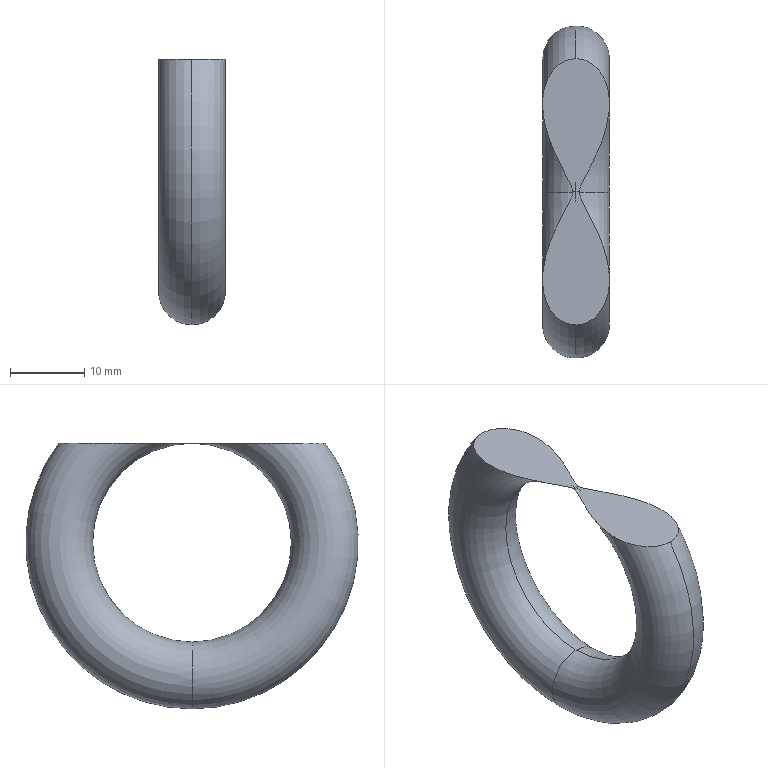Component | SolidWorks | M12LiftingEyeAssembly1-2_M12LiftingEye-1 | 1 solid | 5 faces | box 9 x 44.76 x 35.78 mm | volume 5538 mm3 | torus 4 | plane 1
STEP:
#1=COLOUR_RGB('',0.7922,0.8196,0.9333);
#2=FILL_AREA_STYLE_COLOUR('',#1);
#3=FILL_AREA_STYLE('',(#2));
#4=SURFACE_STYLE_FILL_AREA(#3);
#5=SURFACE_SIDE_STYLE('',(#4));
#6=SURFACE_STYLE_USAGE(.BOTH.,#5);
#7=PRESENTATION_STYLE_ASSIGNMENT((#6));
#8=CARTESIAN_POINT('',(20.866,-0.1144,-0.3588));
#9=VERTEX_POINT('',#8);
#10=CARTESIAN_POINT('',(20.849,-0.82,-0.3588));
#11=VERTEX_POINT('',#10);
#12=CARTESIAN_POINT('',(20.866,-0.1144,-0.3588));
#13=CARTESIAN_POINT('',(20.866,-0.1231,-0.3588));
#14=CARTESIAN_POINT('',(20.868,-0.1314,-0.3588));
#15=CARTESIAN_POINT('',(20.874,-0.1475,-0.3588));
#16=CARTESIAN_POINT('',(20.878,-0.1554,-0.3588));
#17=CARTESIAN_POINT('',(20.889,-0.1786,-0.3588));
#18=CARTESIAN_POINT('',(20.897,-0.1939,-0.3588));
#19=CARTESIAN_POINT('',(20.921,-0.2397,-0.3588));
#20=CARTESIAN_POINT('',(20.937,-0.2703,-0.3588));
#21=CARTESIAN_POINT('',(20.966,-0.3326,-0.3588));
#22=CARTESIAN_POINT('',(20.98,-0.3642,-0.3588));
#23=CARTESIAN_POINT('',(20.997,-0.4127,-0.3588));
#24=CARTESIAN_POINT('',(21.002,-0.4291,-0.3588));
#25=CARTESIAN_POINT('',(21.011,-0.4623,-0.3588));
#26=CARTESIAN_POINT('',(21.015,-0.4792,-0.3588));
#27=CARTESIAN_POINT('',(21.024,-0.5304,-0.3588));
#28=CARTESIAN_POINT('',(21.027,-0.5648,-0.3588));
#29=CARTESIAN_POINT('',(21.025,-0.617,-0.3588));
#30=CARTESIAN_POINT('',(21.023,-0.6341,-0.3588));
#31=CARTESIAN_POINT('',(21.016,-0.6677,-0.3588));
#32=CARTESIAN_POINT('',(21.011,-0.6843,-0.3588));
#33=CARTESIAN_POINT('',(21.001,-0.7085,-0.3588));
#34=CARTESIAN_POINT('',(20.998,-0.7164,-0.3588));
#35=CARTESIAN_POINT('',(20.989,-0.7317,-0.3588));
#36=CARTESIAN_POINT('',(20.985,-0.7391,-0.3588));
#37=CARTESIAN_POINT('',(20.97,-0.7604,-0.3588));
#38=CARTESIAN_POINT('',(20.958,-0.7735,-0.3588));
#39=CARTESIAN_POINT('',(20.938,-0.79,-0.3588));
#40=CARTESIAN_POINT('',(20.931,-0.795,-0.3588));
#41=CARTESIAN_POINT('',(20.916,-0.8038,-0.3588));
#42=CARTESIAN_POINT('',(20.908,-0.8076,-0.3588));
#43=CARTESIAN_POINT('',(20.892,-0.8137,-0.3588));
#44=CARTESIAN_POINT('',(20.883,-0.816,-0.3588));
#45=CARTESIAN_POINT('',(20.866,-0.8192,-0.3588));
#46=CARTESIAN_POINT('',(20.858,-0.82,-0.3588));
#47=CARTESIAN_POINT('',(20.849,-0.82,-0.3588));
#48=B_SPLINE_CURVE_WITH_KNOTS('',3,(#12,#13,#14,#15,#16,#17,#18,#19,#20,#21,#22,#23,#24,#25,#26,#27,#28,#29,#30,#31,#32,#33,#34,#35,#36,#37,#38,#39,#40,#41,#42,#43,#44,#45,#46,#47),.UNSPECIFIED.,.F.,.F.,(4,2,2,2,2,2,2,2,2,2,2,2,2,2,2,2,2,4),(0.,0.0006517,0.001303,0.002607,0.005214,0.007821,0.009124,0.01043,0.01303,0.01434,0.01564,0.01629,0.01694,0.01825,0.0189,0.01955,0.0202,0.02086),.UNSPECIFIED.);
#49=EDGE_CURVE('',#9,#11,#48,.T.);
#50=ORIENTED_EDGE('',*,*,#49,.T.);
#51=CARTESIAN_POINT('',(20.849,-0.1144,-1.767));
#52=VERTEX_POINT('',#51);
#53=CARTESIAN_POINT('',(20.849,-0.1144,-0.8864));
#54=DIRECTION('',(1.,0.,0.));
#55=DIRECTION('',(0.,0.,-1.));
#56=AXIS2_PLACEMENT_3D('',#53,#54,#55);
#57=CIRCLE('',#56,0.8811);
#58=EDGE_CURVE('',#11,#52,#57,.T.);
#59=ORIENTED_EDGE('',*,*,#58,.T.);
#60=CARTESIAN_POINT('',(20.849,-0.1144,-1.413));
#61=VERTEX_POINT('',#60);
#62=CARTESIAN_POINT('',(20.849,-0.1144,-1.59));
#63=DIRECTION('',(0.,-1.,0.));
#64=DIRECTION('',(0.,0.,-1.));
#65=AXIS2_PLACEMENT_3D('',#62,#63,#64);
#66=CIRCLE('',#65,0.1772);
#67=EDGE_CURVE('',#52,#61,#66,.T.);
#68=ORIENTED_EDGE('',*,*,#67,.T.);
#69=CARTESIAN_POINT('',(20.849,-0.1144,-0.3596));
#70=VERTEX_POINT('',#69);
#71=CARTESIAN_POINT('',(20.849,-0.1144,-0.8864));
#72=DIRECTION('',(1.,0.,0.));
#73=DIRECTION('',(0.,0.,-1.));
#74=AXIS2_PLACEMENT_3D('',#71,#72,#73);
#75=CIRCLE('',#74,0.5267);
#76=EDGE_CURVE('',#70,#61,#75,.T.);
#77=ORIENTED_EDGE('',*,*,#76,.F.);
#78=CARTESIAN_POINT('',(20.849,-0.1144,-0.1825));
#79=DIRECTION('',(0.,1.,-0.));
#80=DIRECTION('',(0.,0.,1.));
#81=AXIS2_PLACEMENT_3D('',#78,#79,#80);
#82=CIRCLE('',#81,0.1772);
#83=EDGE_CURVE('',#9,#70,#82,.T.);
#84=ORIENTED_EDGE('',*,*,#83,.F.);
#85=EDGE_LOOP('',(#50,#59,#68,#77,#84));
#86=FACE_OUTER_BOUND('',#85,.T.);
#87=CARTESIAN_POINT('',(20.849,-0.1144,-0.8864));
#88=DIRECTION('',(1.,0.,0.));
#89=DIRECTION('',(0.,0.,-1.));
#90=AXIS2_PLACEMENT_3D('',#87,#88,#89);
#91=TOROIDAL_SURFACE('',#90,0.7039,0.1772);
#92=ADVANCED_FACE('',(#86),#91,.T.);
#93=ORIENTED_EDGE('',*,*,#67,.F.);
#94=CARTESIAN_POINT('',(20.849,0.5913,-0.3588));
#95=VERTEX_POINT('',#94);
#96=CARTESIAN_POINT('',(20.849,-0.1144,-0.8864));
#97=DIRECTION('',(1.,0.,0.));
#98=DIRECTION('',(0.,0.,-1.));
#99=AXIS2_PLACEMENT_3D('',#96,#97,#98);
#100=CIRCLE('',#99,0.8811);
#101=EDGE_CURVE('',#52,#95,#100,.T.);
#102=ORIENTED_EDGE('',*,*,#101,.T.);
#103=CARTESIAN_POINT('',(20.849,0.5913,-0.3588));
#104=CARTESIAN_POINT('',(20.858,0.5913,-0.3588));
#105=CARTESIAN_POINT('',(20.866,0.5905,-0.3588));
#106=CARTESIAN_POINT('',(20.883,0.5873,-0.3588));
#107=CARTESIAN_POINT('',(20.892,0.585,-0.3588));
#108=CARTESIAN_POINT('',(20.908,0.5788,-0.3588));
#109=CARTESIAN_POINT('',(20.916,0.5751,-0.3588));
#110=CARTESIAN_POINT('',(20.931,0.5663,-0.3588));
#111=CARTESIAN_POINT('',(20.938,0.5613,-0.3588));
#112=CARTESIAN_POINT('',(20.958,0.5447,-0.3588));
#113=CARTESIAN_POINT('',(20.97,0.5319,-0.3588));
#114=CARTESIAN_POINT('',(20.99,0.5032,-0.3588));
#115=CARTESIAN_POINT('',(20.998,0.4879,-0.3588));
#116=CARTESIAN_POINT('',(21.011,0.456,-0.3588));
#117=CARTESIAN_POINT('',(21.016,0.4391,-0.3588));
#118=CARTESIAN_POINT('',(21.023,0.4053,-0.3588));
#119=CARTESIAN_POINT('',(21.025,0.3883,-0.3588));
#120=CARTESIAN_POINT('',(21.026,0.3539,-0.3588));
#121=CARTESIAN_POINT('',(21.026,0.3365,-0.3588));
#122=CARTESIAN_POINT('',(21.023,0.302,-0.3588));
#123=CARTESIAN_POINT('',(21.021,0.285,-0.3588));
#124=CARTESIAN_POINT('',(21.012,0.2344,-0.3588));
#125=CARTESIAN_POINT('',(21.003,0.2014,-0.3588));
#126=CARTESIAN_POINT('',(20.98,0.1362,-0.3588));
#127=CARTESIAN_POINT('',(20.967,0.1044,-0.3588));
#128=CARTESIAN_POINT('',(20.937,0.04187,-0.3588));
#129=CARTESIAN_POINT('',(20.922,0.01119,-0.3588));
#130=CARTESIAN_POINT('',(20.897,-0.03467,-0.3588));
#131=CARTESIAN_POINT('',(20.889,-0.04991,-0.3588));
#132=CARTESIAN_POINT('',(20.878,-0.07319,-0.3588));
#133=CARTESIAN_POINT('',(20.874,-0.08103,-0.3588));
#134=CARTESIAN_POINT('',(20.868,-0.09715,-0.3588));
#135=CARTESIAN_POINT('',(20.866,-0.1056,-0.3588));
#136=CARTESIAN_POINT('',(20.866,-0.1144,-0.3588));
#137=B_SPLINE_CURVE_WITH_KNOTS('',3,(#103,#104,#105,#106,#107,#108,#109,#110,#111,#112,#113,#114,#115,#116,#117,#118,#119,#120,#121,#122,#123,#124,#125,#126,#127,#128,#129,#130,#131,#132,#133,#134,#135,#136),.UNSPECIFIED.,.F.,.F.,(4,2,2,2,2,2,2,2,2,2,2,2,2,2,2,2,4),(0.06255,0.06321,0.06386,0.06451,0.06516,0.06647,0.06777,0.06908,0.07038,0.07169,0.07299,0.0756,0.07821,0.08082,0.08213,0.08278,0.08343),.UNSPECIFIED.);
#138=EDGE_CURVE('',#95,#9,#137,.T.);
#139=ORIENTED_EDGE('',*,*,#138,.T.);
#140=ORIENTED_EDGE('',*,*,#83,.T.);
#141=CARTESIAN_POINT('',(20.849,-0.1144,-0.8864));
#142=DIRECTION('',(1.,0.,0.));
#143=DIRECTION('',(0.,0.,-1.));
#144=AXIS2_PLACEMENT_3D('',#141,#142,#143);
#145=CIRCLE('',#144,0.5267);
#146=EDGE_CURVE('',#61,#70,#145,.T.);
#147=ORIENTED_EDGE('',*,*,#146,.F.);
#148=EDGE_LOOP('',(#93,#102,#139,#140,#147));
#149=FACE_OUTER_BOUND('',#148,.T.);
#150=CARTESIAN_POINT('',(20.849,-0.1144,-0.8864));
#151=DIRECTION('',(1.,0.,0.));
#152=DIRECTION('',(0.,0.,-1.));
#153=AXIS2_PLACEMENT_3D('',#150,#151,#152);
#154=TOROIDAL_SURFACE('',#153,0.7039,0.1772);
#155=ADVANCED_FACE('',(#149),#154,.T.);
#156=ORIENTED_EDGE('',*,*,#101,.F.);
#157=CARTESIAN_POINT('',(20.849,-0.1144,-1.59));
#158=DIRECTION('',(0.,-1.,0.));
#159=DIRECTION('',(0.,0.,-1.));
#160=AXIS2_PLACEMENT_3D('',#157,#158,#159);
#161=CIRCLE('',#160,0.1772);
#162=EDGE_CURVE('',#61,#52,#161,.T.);
#163=ORIENTED_EDGE('',*,*,#162,.F.);
#164=ORIENTED_EDGE('',*,*,#146,.T.);
#165=CARTESIAN_POINT('',(20.832,-0.1144,-0.3588));
#166=VERTEX_POINT('',#165);
#167=CARTESIAN_POINT('',(20.849,-0.1144,-0.1825));
#168=DIRECTION('',(0.,1.,-0.));
#169=DIRECTION('',(0.,0.,1.));
#170=AXIS2_PLACEMENT_3D('',#167,#168,#169);
#171=CIRCLE('',#170,0.1772);
#172=EDGE_CURVE('',#70,#166,#171,.T.);
#173=ORIENTED_EDGE('',*,*,#172,.T.);
#174=CARTESIAN_POINT('',(20.832,-0.1144,-0.3588));
#175=CARTESIAN_POINT('',(20.832,-0.1057,-0.3588));
#176=CARTESIAN_POINT('',(20.829,-0.09719,-0.3588));
#177=CARTESIAN_POINT('',(20.823,-0.08105,-0.3588));
#178=CARTESIAN_POINT('',(20.82,-0.07326,-0.3588));
#179=CARTESIAN_POINT('',(20.808,-0.05005,-0.3588));
#180=CARTESIAN_POINT('',(20.8,-0.03484,-0.3588));
#181=CARTESIAN_POINT('',(20.776,0.01094,-0.3588));
#182=CARTESIAN_POINT('',(20.76,0.04154,-0.3588));
#183=CARTESIAN_POINT('',(20.731,0.1039,-0.3588));
#184=CARTESIAN_POINT('',(20.718,0.1356,-0.3588));
#185=CARTESIAN_POINT('',(20.701,0.1844,-0.3588));
#186=CARTESIAN_POINT('',(20.696,0.201,-0.3588));
#187=CARTESIAN_POINT('',(20.687,0.2343,-0.3588));
#188=CARTESIAN_POINT('',(20.683,0.2511,-0.3588));
#189=CARTESIAN_POINT('',(20.676,0.285,-0.3588));
#190=CARTESIAN_POINT('',(20.674,0.3021,-0.3588));
#191=CARTESIAN_POINT('',(20.672,0.3366,-0.3588));
#192=CARTESIAN_POINT('',(20.671,0.354,-0.3588));
#193=CARTESIAN_POINT('',(20.673,0.3884,-0.3588));
#194=CARTESIAN_POINT('',(20.675,0.4055,-0.3588));
#195=CARTESIAN_POINT('',(20.682,0.4393,-0.3588));
#196=CARTESIAN_POINT('',(20.687,0.4562,-0.3588));
#197=CARTESIAN_POINT('',(20.7,0.4881,-0.3588));
#198=CARTESIAN_POINT('',(20.708,0.5035,-0.3588));
#199=CARTESIAN_POINT('',(20.728,0.5321,-0.3588));
#200=CARTESIAN_POINT('',(20.74,0.5449,-0.3588));
#201=CARTESIAN_POINT('',(20.76,0.5614,-0.3588));
#202=CARTESIAN_POINT('',(20.767,0.5664,-0.3588));
#203=CARTESIAN_POINT('',(20.782,0.5751,-0.3588));
#204=CARTESIAN_POINT('',(20.79,0.5789,-0.3588));
#205=CARTESIAN_POINT('',(20.806,0.585,-0.3588));
#206=CARTESIAN_POINT('',(20.815,0.5874,-0.3588));
#207=CARTESIAN_POINT('',(20.832,0.5905,-0.3588));
#208=CARTESIAN_POINT('',(20.84,0.5913,-0.3588));
#209=CARTESIAN_POINT('',(20.849,0.5913,-0.3588));
#210=B_SPLINE_CURVE_WITH_KNOTS('',3,(#174,#175,#176,#177,#178,#179,#180,#181,#182,#183,#184,#185,#186,#187,#188,#189,#190,#191,#192,#193,#194,#195,#196,#197,#198,#199,#200,#201,#202,#203,#204,#205,#206,#207,#208,#209),.UNSPECIFIED.,.F.,.F.,(4,2,2,2,2,2,2,2,2,2,2,2,2,2,2,2,2,4),(0.04165,0.04231,0.04296,0.04427,0.04688,0.04949,0.0508,0.0521,0.05341,0.05472,0.05602,0.05733,0.05863,0.05994,0.06059,0.06125,0.0619,0.06255),.UNSPECIFIED.);
#211=EDGE_CURVE('',#166,#95,#210,.T.);
#212=ORIENTED_EDGE('',*,*,#211,.T.);
#213=EDGE_LOOP('',(#156,#163,#164,#173,#212));
#214=FACE_OUTER_BOUND('',#213,.T.);
#215=CARTESIAN_POINT('',(20.849,-0.1144,-0.8864));
#216=DIRECTION('',(1.,0.,0.));
#217=DIRECTION('',(0.,0.,-1.));
#218=AXIS2_PLACEMENT_3D('',#215,#216,#217);
#219=TOROIDAL_SURFACE('',#218,0.7039,0.1772);
#220=ADVANCED_FACE('',(#214),#219,.T.);
#221=ORIENTED_EDGE('',*,*,#58,.F.);
#222=CARTESIAN_POINT('',(20.849,-0.82,-0.3588));
#223=CARTESIAN_POINT('',(20.84,-0.82,-0.3588));
#224=CARTESIAN_POINT('',(20.832,-0.8192,-0.3588));
#225=CARTESIAN_POINT('',(20.814,-0.8161,-0.3588));
#226=CARTESIAN_POINT('',(20.806,-0.8137,-0.3588));
#227=CARTESIAN_POINT('',(20.782,-0.8045,-0.3588));
#228=CARTESIAN_POINT('',(20.766,-0.7955,-0.3588));
#229=CARTESIAN_POINT('',(20.74,-0.7736,-0.3588));
#230=CARTESIAN_POINT('',(20.728,-0.7604,-0.3588));
#231=CARTESIAN_POINT('',(20.708,-0.7321,-0.3588));
#232=CARTESIAN_POINT('',(20.7,-0.7168,-0.3588));
#233=CARTESIAN_POINT('',(20.687,-0.6845,-0.3588));
#234=CARTESIAN_POINT('',(20.682,-0.668,-0.3588));
#235=CARTESIAN_POINT('',(20.675,-0.6343,-0.3588));
#236=CARTESIAN_POINT('',(20.673,-0.617,-0.3588));
#237=CARTESIAN_POINT('',(20.67,-0.5651,-0.3588));
#238=CARTESIAN_POINT('',(20.673,-0.5309,-0.3588));
#239=CARTESIAN_POINT('',(20.683,-0.4801,-0.3588));
#240=CARTESIAN_POINT('',(20.686,-0.4631,-0.3588));
#241=CARTESIAN_POINT('',(20.696,-0.4298,-0.3588));
#242=CARTESIAN_POINT('',(20.701,-0.4134,-0.3588));
#243=CARTESIAN_POINT('',(20.718,-0.3647,-0.3588));
#244=CARTESIAN_POINT('',(20.731,-0.333,-0.3588));
#245=CARTESIAN_POINT('',(20.76,-0.2705,-0.3588));
#246=CARTESIAN_POINT('',(20.776,-0.2398,-0.3588));
#247=CARTESIAN_POINT('',(20.8,-0.1939,-0.3588));
#248=CARTESIAN_POINT('',(20.808,-0.1787,-0.3588));
#249=CARTESIAN_POINT('',(20.82,-0.1554,-0.3588));
#250=CARTESIAN_POINT('',(20.823,-0.1476,-0.3588));
#251=CARTESIAN_POINT('',(20.828,-0.1355,-0.3588));
#252=CARTESIAN_POINT('',(20.829,-0.1314,-0.3588));
#253=CARTESIAN_POINT('',(20.831,-0.123,-0.3588));
#254=CARTESIAN_POINT('',(20.832,-0.1186,-0.3588));
#255=CARTESIAN_POINT('',(20.832,-0.1144,-0.3588));
#256=B_SPLINE_CURVE_WITH_KNOTS('',3,(#222,#223,#224,#225,#226,#227,#228,#229,#230,#231,#232,#233,#234,#235,#236,#237,#238,#239,#240,#241,#242,#243,#244,#245,#246,#247,#248,#249,#250,#251,#252,#253,#254,#255),.UNSPECIFIED.,.F.,.F.,(4,2,2,2,2,2,2,2,2,2,2,2,2,2,2,2,4),(0.02086,0.0215,0.02215,0.02345,0.02475,0.02605,0.02735,0.02865,0.03125,0.03255,0.03385,0.03645,0.03905,0.04035,0.041,0.04133,0.04165),.UNSPECIFIED.);
#257=EDGE_CURVE('',#11,#166,#256,.T.);
#258=ORIENTED_EDGE('',*,*,#257,.T.);
#259=ORIENTED_EDGE('',*,*,#172,.F.);
#260=ORIENTED_EDGE('',*,*,#76,.T.);
#261=ORIENTED_EDGE('',*,*,#162,.T.);
#262=EDGE_LOOP('',(#221,#258,#259,#260,#261));
#263=FACE_OUTER_BOUND('',#262,.T.);
#264=CARTESIAN_POINT('',(20.849,-0.1144,-0.8864));
#265=DIRECTION('',(1.,0.,0.));
#266=DIRECTION('',(0.,0.,-1.));
#267=AXIS2_PLACEMENT_3D('',#264,#265,#266);
#268=TOROIDAL_SURFACE('',#267,0.7039,0.1772);
#269=ADVANCED_FACE('',(#263),#268,.T.);
#270=ORIENTED_EDGE('',*,*,#49,.F.);
#271=ORIENTED_EDGE('',*,*,#138,.F.);
#272=ORIENTED_EDGE('',*,*,#211,.F.);
#273=ORIENTED_EDGE('',*,*,#257,.F.);
#274=EDGE_LOOP('',(#270,#271,#272,#273));
#275=FACE_OUTER_BOUND('',#274,.T.);
#276=CARTESIAN_POINT('',(20.849,-0.1143,-0.3588));
#277=DIRECTION('',(0.,0.,-1.));
#278=DIRECTION('',(-1.,0.,-0.));
#279=AXIS2_PLACEMENT_3D('',#276,#277,#278);
#280=PLANE('',#279);
#281=ADVANCED_FACE('',(#275),#280,.F.);
#282=CLOSED_SHELL('',(#92,#155,#220,#269,#281));
#283=MANIFOLD_SOLID_BREP('',#282);
#284=STYLED_ITEM('',(#7),#283);
#285=PRESENTATION_LAYER_ASSIGNMENT('','',(#284));
#286=CARTESIAN_POINT('',(0.,0.,0.));
#287=DIRECTION('',(0.,0.,1.));
#288=DIRECTION('',(1.,0.,0.));
#289=AXIS2_PLACEMENT_3D('',#286,#287,#288);
#290=(LENGTH_UNIT()NAMED_UNIT(*)SI_UNIT($,.METRE.));
#291=LENGTH_MEASURE_WITH_UNIT(LENGTH_MEASURE(0.0254),#290);
#292=DIMENSIONAL_EXPONENTS(1.,0.,0.,0.,0.,0.,0.);
#293=(CONVERSION_BASED_UNIT('',#291)LENGTH_UNIT()NAMED_UNIT(#292));
#294=UNCERTAINTY_MEASURE_WITH_UNIT(LENGTH_MEASURE(0.00001),#293,'','');
#295=(NAMED_UNIT(*)PLANE_ANGLE_UNIT()SI_UNIT($,.RADIAN.));
#296=(NAMED_UNIT(*)SI_UNIT($,.STERADIAN.)SOLID_ANGLE_UNIT());
#297=(GEOMETRIC_REPRESENTATION_CONTEXT(3)GLOBAL_UNCERTAINTY_ASSIGNED_CONTEXT((#294))GLOBAL_UNIT_ASSIGNED_CONTEXT((#293,#295,#296))REPRESENTATION_CONTEXT('',''));
#298=ADVANCED_BREP_SHAPE_REPRESENTATION('',(#283,#289),#297);
#299=(LENGTH_UNIT()NAMED_UNIT(*)SI_UNIT($,.METRE.));
#300=LENGTH_MEASURE_WITH_UNIT(LENGTH_MEASURE(0.0254),#299);
#301=DIMENSIONAL_EXPONENTS(1.,0.,0.,0.,0.,0.,0.);
#302=(CONVERSION_BASED_UNIT('',#300)LENGTH_UNIT()NAMED_UNIT(#301));
#303=UNCERTAINTY_MEASURE_WITH_UNIT(LENGTH_MEASURE(0.00001),#302,'','');
#304=(NAMED_UNIT(*)PLANE_ANGLE_UNIT()SI_UNIT($,.RADIAN.));
#305=(NAMED_UNIT(*)SI_UNIT($,.STERADIAN.)SOLID_ANGLE_UNIT());
#306=(GEOMETRIC_REPRESENTATION_CONTEXT(3)GLOBAL_UNCERTAINTY_ASSIGNED_CONTEXT((#303))GLOBAL_UNIT_ASSIGNED_CONTEXT((#302,#304,#305))REPRESENTATION_CONTEXT('',''));
#307=MECHANICAL_DESIGN_GEOMETRIC_PRESENTATION_REPRESENTATION('',(#284),#306);